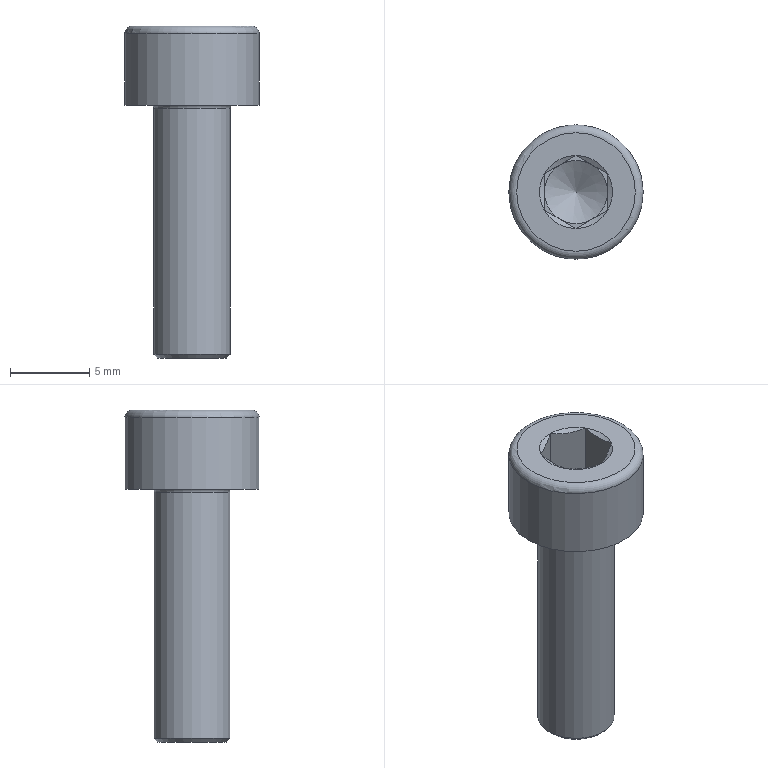Component | NX | GB-T70_1-2000_M5X16 | 1 solid | 27 faces | volume 527 mm3 | plane 15 | cone 8 | cylinder 2 | torus 2 | commonest cylinder face diameters 4.826 x1 8.5 x1